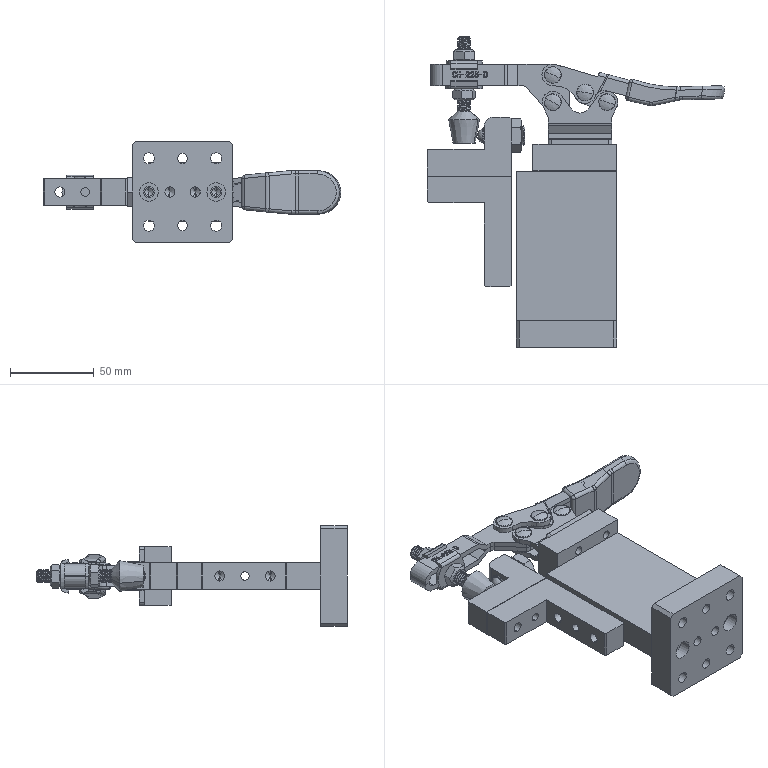Assembly | SolidWorks | mm | 22 component files | 24 solids | 1263 faces | box 177.34 x 185.09 x 60 mm | volume 233117 mm3 | plane 425 | cylinder 407 | spline 224 | cone 179 | torus 26 | sphere 2 | commonest cylinder face diameters 7.92 x72 6 x49 4 x38 6.4 x32 10 x28 6.3 x28 10.2 x21 5 x20
Bill of materials:
AdjustmentSeat001 | 1 | Plain Carbon Steel | L-shaped solid bar block with rectangular cross-section, two perpendicular legs, and round through-holes in the side faces; small chamfers on the outer vertical edges.
225-D-01 | 1 |  | Formed sheet-metal bracket: a flat mounting flange with four obround slots, bent into two parallel offset lugs, each with one round hole. The lug plate outline has two rounded ears and a central V-shaped notch.
225-D-02 | 1 |  | Flat strip bent into a closed elongated loop at one end; the two strip ends are joined into a widened flat tab with two round holes and angled/chamfered corners.
225-D-03 | 1 |  | Forked lever: two parallel thin ears, each with two round holes, join into a solid body that tapers in plan view and ends in a rounded, paddle-like flattened tip.
225-D-04 | 2 |  | Flat obround (stadium-shaped) link plate of uniform thickness with two round through-holes near its ends.
225-D-05 | 4 |  | Cylindrical pin with a domed head at each end; it looks like a rivet or pin with two formed heads.
225-D-06 | 1 |  | Solid rounded lever-grip or paddle shape: a tapered flat body with a semicircular end, a slightly cranked/curved profile, and filleted edges all round.
56212-01 | 2 |  | Hexagonal nut with an internally threaded central bore and chamfered corners on both faces.
CH-FC-56212 | 1 |  | Threaded screw or stud with a smooth conical (frustum) head and no visible drive recess; a long threaded shank runs to a slightly chamfered end.
FW-516 | 2 |  | Formed plate with a round central hole, circular-arc side edges, and two straight opposite edges bent out of plane into short angled flanges.
GB_T6172.1-2000HexagonThinNutAAndBM12 | 1 |  | Thin hexagonal nut (low height relative to width) with a large central bore and chamfered corners.
GB_T77-2000HexagonSocketSetScrewWithFlatPointM12_25 | 1 |  | Headless externally threaded set-screw-like part with a rounded/domed tip at one end and a recessed drive socket in the flat opposite end.
LocatingBlock2-001 | 1 | AISI Type A2 Tool Steel | L-shaped prismatic block of constant thickness. The long arm has a row of three cross holes in its side face, and the end face of the short arm has one larger bore.
QuickClampBackingPlate | 1 | 6061 Alloy | Plain rectangular block with six round holes through one large face: two larger holes on the horizontal centerline and four smaller holes in a rectangular pattern.
UnitFixingPlate001 | 1 | 6061 Alloy | Thick, nearly square plate with all four corners chamfered and ten through holes in three rows.
UnitFixingSeat2-002 | 1 | 6061 Alloy | Rectangular slab with a plain top face. One long side face has a row of four drilled holes, and the adjacent end face has one larger hole.
Mates:
1. distance | AdjustmentSeat001-1 face at (-1.972, 9.101, 125.932) dir (1, 0, 0) | UnitFixingSeat2-002-1 face at (1.028, 28.101, 125.932) dir (-1, 0, 0)
2. coincident | AdjustmentSeat001-1 face at (-17.972, 9.101, 125.932) dir (0, 0, 1) | UnitFixingSeat2-002-1 face at (31.028, -16.399, 125.932) dir (0, 0, 1)
3. distance | AdjustmentSeat001-1 face at (-1.972, -40.899, 125.932) dir (0, -1, 0) | UnitFixingSeat2-002-1 face at (61.028, -60.899, 125.932) dir (0, -1, 0)
4. coincident | UnitFixingSeat2-002-1 face at (61.028, -60.899, 125.932) dir (0, -1, 0) | UnitFixingPlate001-1 face at (31.028, -60.899, 117.932) dir (0, 1, 0)
5. coincident | UnitFixingSeat2-002-1 face at (61.028, 28.101, 125.932) dir (1, 0, 0) | UnitFixingPlate001-1 face at (61.028, -60.899, 87.932) dir (1, 0, 0)
6. coincident | UnitFixingSeat2-002-1 plane at (31.028, -16.399, 117.932) dir (0, 0, 1) | UnitFixingPlate001-1 plane at (31.028, -68.899, 117.932) dir (0, 0, -1)
7. distance | UnitFixingSeat2-002-1 face at (61.028, 28.101, 125.932) dir (0, 1, 0) | CH-225-D-1/225-D-01-1 face at (20.028, 44.101, 120.932) dir (0, -1, 0)
8. distance | CH-225-D-1/225-D-01-1 face at (61.849, 56.604, 123.932) dir (0, 0, 1) | UnitFixingSeat2-002-1 face at (31.028, -16.399, 125.932) dir (0, 0, 1)
9. distance | UnitFixingSeat2-002-1 face at (61.028, 28.101, 125.932) dir (1, 0, 0) | CH-225-D-1/225-D-01-1 face at (58.028, 44.101, 117.932) dir (1, 0, 0)
10. coincident | UnitFixingSeat2-002-1 face at (61.028, 28.101, 125.932) dir (0, 1, 0) | QuickClampBackingPlate-1 face at (36.028, 28.101, 117.932) dir (0, -1, 0)
11. coincident | UnitFixingSeat2-002-1 face at (61.028, 28.101, 125.932) dir (1, 0, 0) | QuickClampBackingPlate-1 face at (61.028, 28.101, 135.432) dir (1, 0, 0)
12. coincident | UnitFixingSeat2-002-1 plane at (31.028, -16.399, 117.932) dir (0, 0, 1) | QuickClampBackingPlate-1 plane at (36.028, 36.101, 117.932) dir (0, 0, 1)
13. coincident | AdjustmentSeat001-1 face at (-17.972, 25.101, 125.932) dir (0, 1, 0) | LocatingBlock2-001-1 face at (-1.972, 25.101, 125.932) dir (0, -1, 0)
14. concentric | AdjustmentSeat001-1 face at (-26.972, 25.101, 117.932) dir (0, 1, 0) r 2.5 | LocatingBlock2-001-1 face at (-26.972, 41.101, 117.932) dir (0, 1, 0) r 5.5
15. coincident | AdjustmentSeat001-1 face at (-17.972, 9.101, 125.932) dir (0, 0, 1) | LocatingBlock2-001-1 face at (-1.972, 25.101, 125.932) dir (0, 0, 1)
16. concentric | LocatingBlock2-001-1 face at (-17.972, 49.101, 117.932) dir (-1, 0, 0) r 5.1 | GB_T77-2000HexagonSocketSetScrewWithFlatPointM12_25-1 face at (-18.392, 49.101, 117.932) dir (1, 0, 0) r 1042.507
17. distance | GB_T77-2000HexagonSocketSetScrewWithFlatPointM12_25-1 face at (6.028, 45.722, 113.986) dir (1, 0, 0) | LocatingBlock2-001-1 face at (-1.972, 60.101, 125.932) dir (1, 0, 0)
18. coincident | LocatingBlock2-001-1 face at (-1.972, 60.101, 125.932) dir (1, 0, 0) | GB_T6172.1-2000HexagonThinNutAAndBM12-1 face at (-1.972, 54.074, 126.625) dir (-1, 0, 0)
19. coincident | GB_T77-2000HexagonSocketSetScrewWithFlatPointM12_25-1 edge at (5.224, 49.101, 117.932) dir (-1, 0, 0) r 6 | GB_T6172.1-2000HexagonThinNutAAndBM12-1 face at (-1.972, 49.101, 117.932) dir (1, 0, 0) r 6
20. coincident | 225-D-03-1 face at (79.177, 11.14, -11.25) dir (0.02463, -0.9997, 0) | 225-D-06-1 face at (85.714, 11.301, -11.25) dir (-0.02463, 0.9997, 0)
21. coincident | 225-D-03-1 face at (40.796, 8.614, 10.75) dir (0, 0, 1) | 225-D-06-1 face at (57.605, 10.555, 10.75) dir (0, 0, -1)